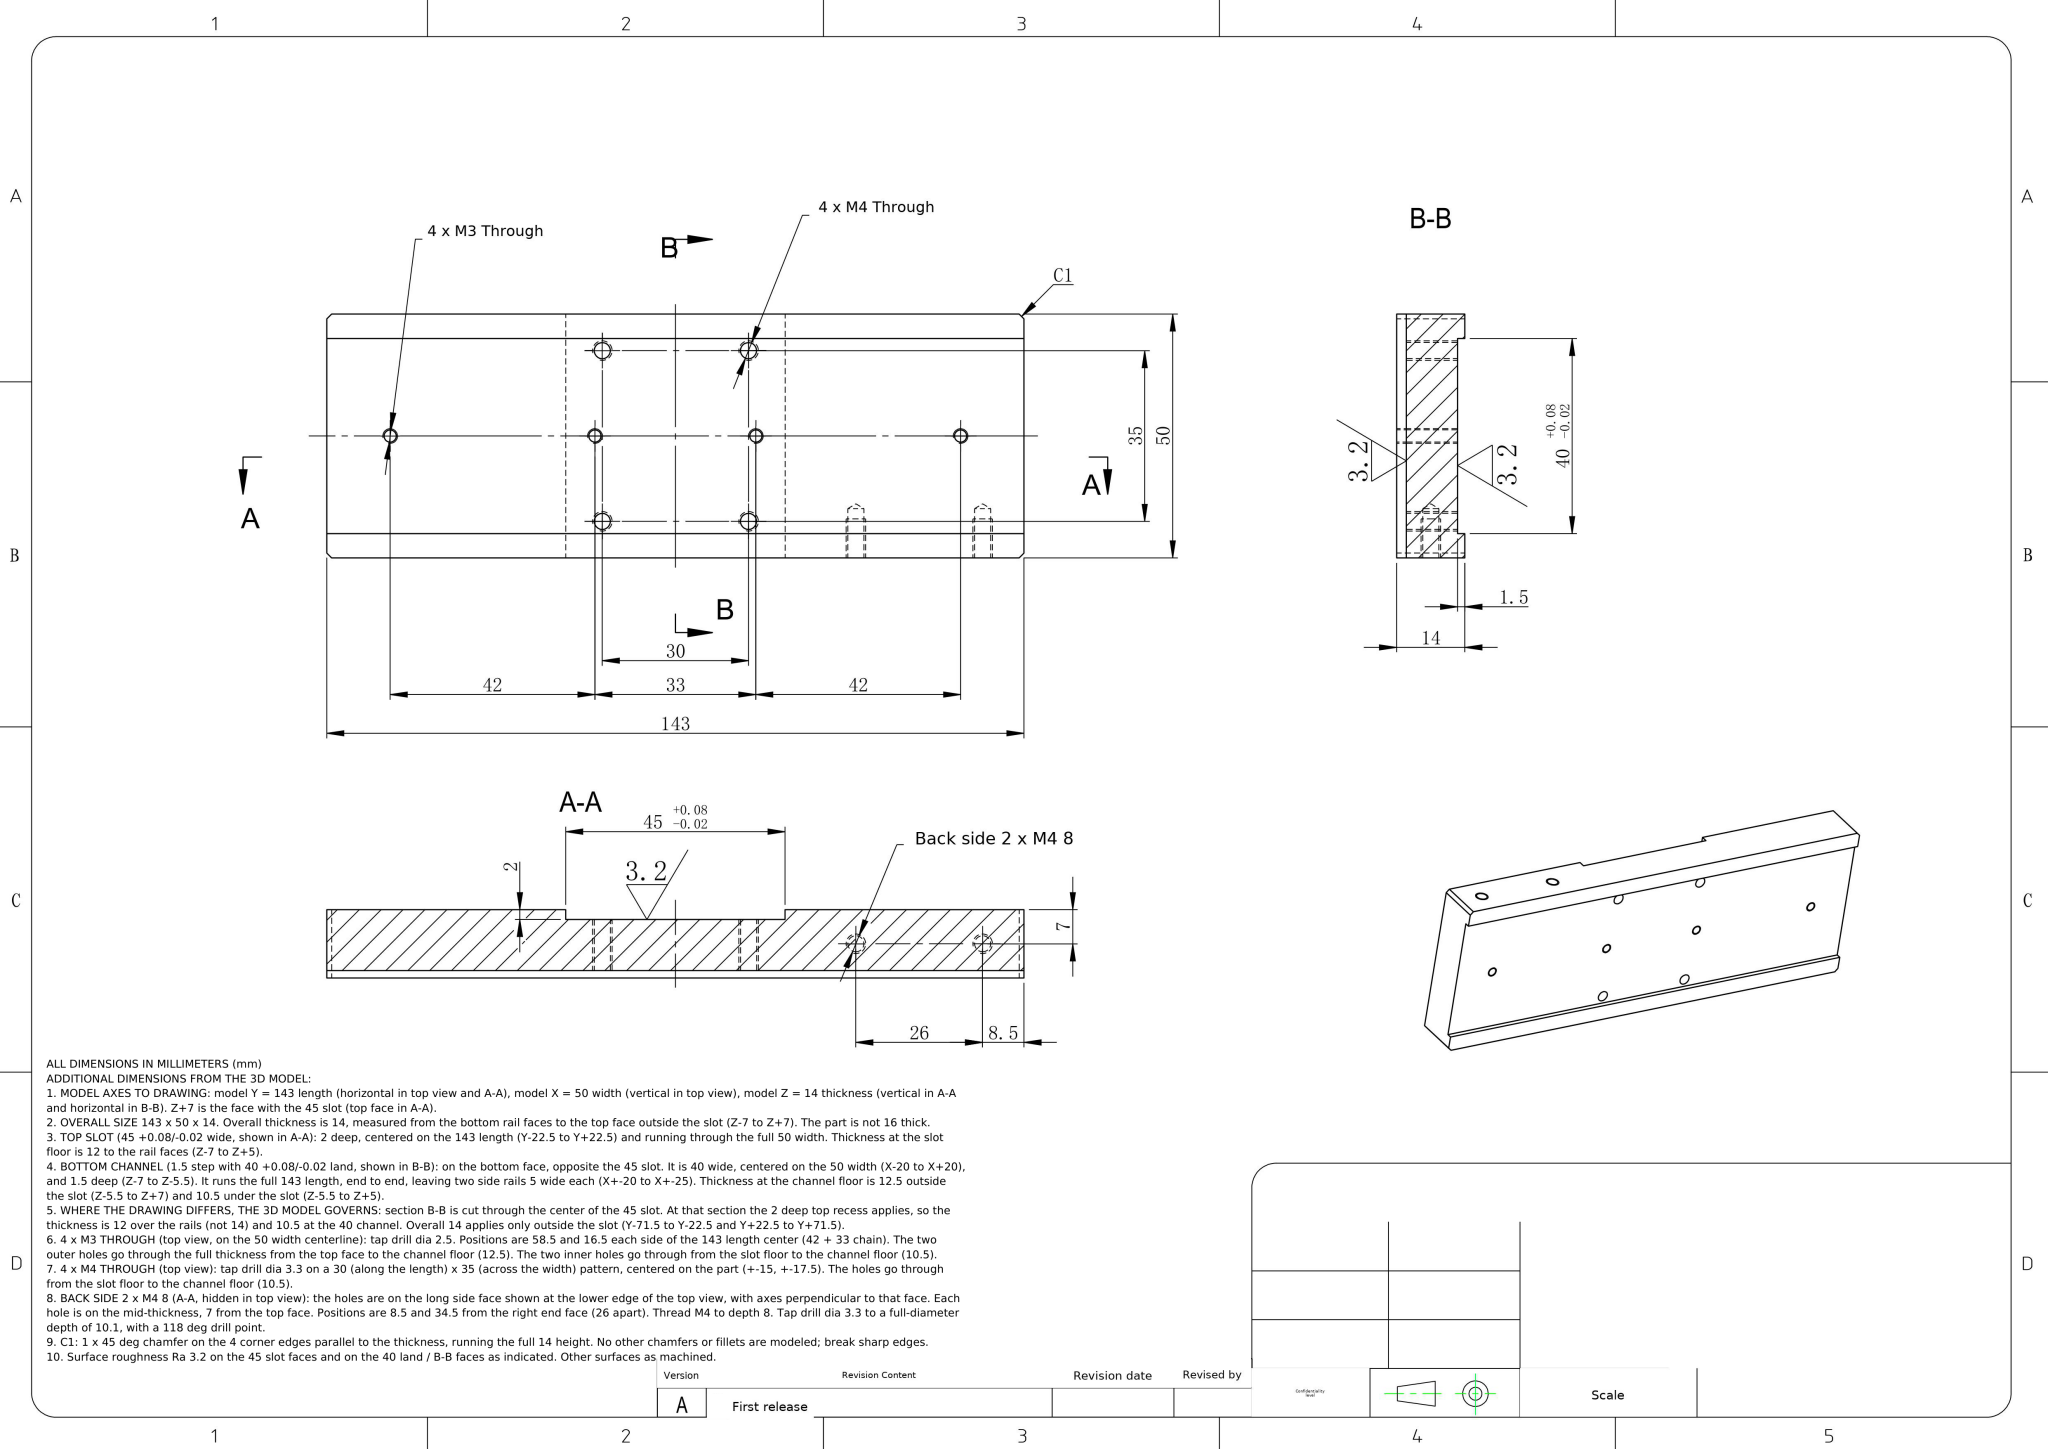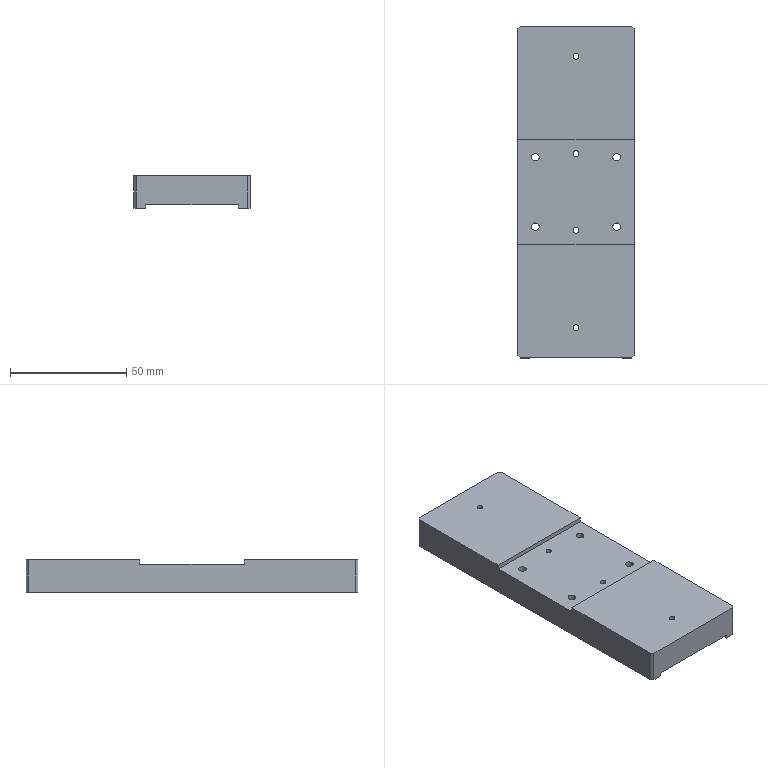Part | NX | mm | Stepped Multi-Bore Adapter Plate 143mm | 1 solid | 42 faces | box 50 x 143 x 14 mm | volume 86229 mm3 | cylinder 20 | plane 18 | cone 4 | commonest cylinder face diameters 3.3 x12 2.5 x8